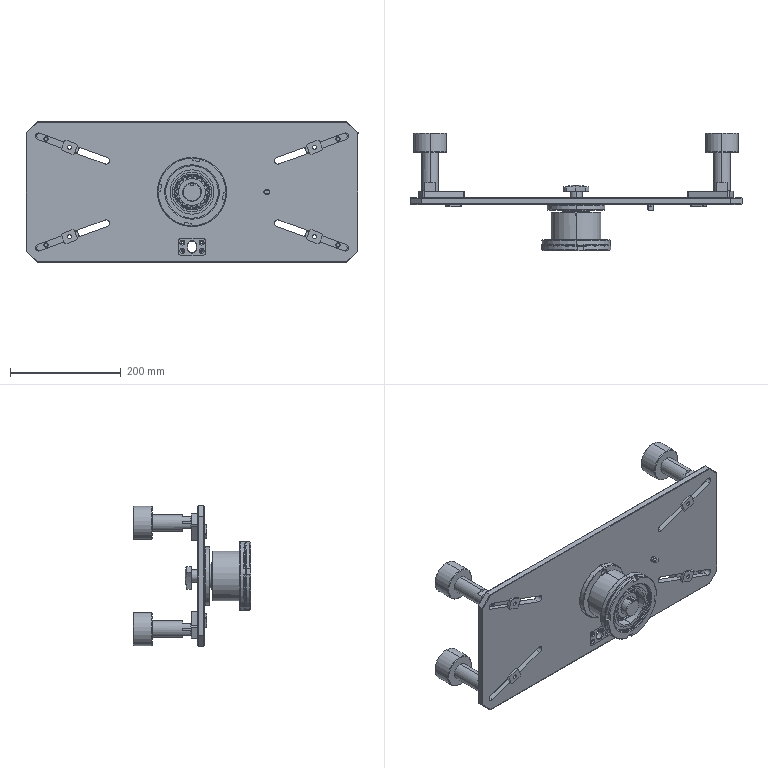Assembly | SolidWorks | mm | 30 component files | 30 solids | 1128 faces | box 600 x 213 x 255 mm | volume 2843561 mm3 | plane 427 | cone 266 | cylinder 261 | torus 164 | spline 10 | commonest cylinder face diameters 10 x25 8.5 x20 15 x16 8 x16 6.8 x16 12 x12 6 x9 16 x9
Bill of materials:
JBH10-8 | 2 | '- | Flanged cylindrical sleeve with a plain through bore; a short, wider flange at one end and a longer, smaller-diameter shank.
MA060.03.03-01 | 1 | AL5052 | Thin flat rectangular plate with chamfered corners, four long slots angled toward the corners, and a central group of round holes.
MA060.03.03-02 | 1 | 45# | Stepped turned pin: a small-diameter spigot, a larger cylindrical body, and a tapered conical nose with a rounded end.
MA060.03.03-03 | 1 | 45# | Flanged hub sleeve: a round flange with six bolt-circle holes, a large central bore with two opposite keyway-like notches, and a cylindrical sleeve with a small V-notch at its end.
MA060.03.03-04 | 1 | 45# | Flanged stub shaft: a round flange with holes, short bosses on both faces, and a stepped shaft with a groove and an end slot or keyway.
MA060.03.03-05 | 1 | 45# | Hexagonal-bodied stepped stud: a small cylindrical spigot with a bore, a hexagonal body, and a tapered, rounded nose.
MA060.03.03-06 | 4 | Q235A | Elongated rectangular bar with chamfered corners, two round through holes, and a stepped (offset-layer) cross-section.
MA060.03.03-07 | 4 | Q235A | Small rectangular block with chamfered corners, a single central through hole, and a stepped, two-tier profile.
MA060.03.03-08 | 1 | H68 | Rectangular flange plate with rounded corners, four countersunk holes, and a central obround opening surrounded by a raised obround boss.
MA060.03.03-09 | 1 | Q235A | Cylindrical pin with two parallel flats machined along part of its length, forming a reduced flat-sided end section.
MA060.03.03-10 | 4 | Polyurethane | Solid cylindrical disc or spacer with a small central through hole and chamfered edges.
MA060.03.03-11 | 4 | Chrome Plated Round Bar | Stepped cylindrical pin: a large cylindrical body with a flat-sided reduced section at one end and a small-diameter pin projecting from that end.
NTM10-30 | 1 | '- | Hand-knob-like part: three-lobed head with concave sides and a slightly domed top face, with a cylindrical shoulder and then a smaller plain cylindrical shank with a chamfered end, all on one axis.
small round nuts gb | 1 |  | Thin flat annular ring with four evenly spaced rectangular notches around the outside and chamfered edges; looks like a slotted ring nut.
tab washers for round nut gb | 1 |  | Thin washer-like ring with one inward rectangular tab and six outward rectangular tabs in two groups of three. The outer tabs are bent out of the plane of the ring at different angles. It looks like a tab-style locking washer.
tapered roller bearings gb | 2 |  | Rolling-element bearing-like assembly: an outer ring and an inner ring with a ring of round rolling elements packed closely between them. The inner ring sticks out past the outer ring on one face.
Mates:
1. coincident | MA060.03.03-03-1 plane at (0, 0, 0) dir (0, 0, 1) | assembly plane at (0, 0, 0) dir (0, 0, 1)
2. coincident | MA060.03.03-03-1 plane at (0, 0, 0) dir (0, 1, 0) | assembly plane at (0, 0, 0) dir (0, 1, 0)
3. coincident | MA060.03.03-03-1 plane at (0, 0, 0) dir (1, 0, 0) | assembly plane at (0, 0, 0) dir (1, 0, 0)
4. concentric | MA060.03.03-04-1 face at (0, 80.553, 0) dir (0, -1, 0) r 25 | MA060.03.03-01-1 face at (0, 81.053, 0) dir (0, -1, 0) r 25
5. coincident | MA060.03.03-04-1 face at (0, 78.053, 0) dir (0, 1, 0) | MA060.03.03-01-1 face at (0, 78.053, 0) dir (0, -1, 0)
6. concentric | MA060.03.03-01-1 face at (0, 78.053, -99) dir (0, 1, 0) r 12.5 | MA060.03.03-08-1 face at (0, 90.053, -99) dir (0, -1, 0) r 12.5
7. coincident | MA060.03.03-01-1 face at (0, 83.053, 0) dir (0, -1, 0) | MA060.03.03-08-1 face at (0, 83.053, -99) dir (0, 1, 0)
8. concentric | MA060.03.03-01-1 face at (17.5, 83.053, -106.5) dir (0, -1, 0) r 1.65 | MA060.03.03-08-1 face at (17.5, 78.053, -106.5) dir (0, -1, 0) r 2.25
9. parallel | MA060.03.03-01-1 face at (300, 78.053, -127.5) dir (0, 0, -1) | assembly plane at (0, 0, 0) dir (0, 0, 1)
10. coincident | MA060.03.03-01-1 face at (-275.157, 78.053, -106.534) dir (-0.342, 0, 0.9397) | MA060.03.03-06-2 face at (-278.591, 87.053, -107.784) dir (0.342, 0, -0.9397)
11. coincident | MA060.03.03-01-1 face at (0, 90.053, 0) dir (0, 1, 0) | MA060.03.03-06-2 face at (-276.35, 90.053, -113.939) dir (0, -1, 0)
12. concentric | MA060.03.03-07-9 face at (-221.425, 74.053, -80.645) dir (0, -1, 0) r 3.4 | MA060.03.03-06-2 face at (-221.425, 87.053, -80.645) dir (0, 1, 0) r 4.25
13. coincident | MA060.03.03-01-1 face at (0, 78.053, 0) dir (0, -1, 0) | MA060.03.03-07-9 face at (-213.099, 78.053, -66.973) dir (0, 1, 0)
14. parallel | MA060.03.03-01-1 face at (-275.157, 78.053, -106.534) dir (-0.342, 0, 0.9397) | MA060.03.03-07-9 face at (-213.099, 74.053, -66.973) dir (-0.342, 0, 0.9397)
15. concentric | MA060.03.03-01-1 face at (-41, 90.053, 0) dir (0, 1, 0) r 7.5 | JBH10-8-1 face at (-41, 85.753, 0) dir (0, 1, 0) r 7.5
16. coincident | MA060.03.03-01-1 face at (-41, 82.253, 0) dir (0, -1, 0) | JBH10-8-1 face at (-49.75, 82.253, 0) dir (0, 1, 0)
17. concentric | MA060.03.03-04-1 face at (-41, 72.053, 0) dir (0, 1, 0) r 3 | MA060.03.03-02-1 face at (-41, 73.053, 0) dir (0, -1, 0) r 3
18. coincident | MA060.03.03-04-1 face at (0, 78.053, 0) dir (0, 1, 0) | MA060.03.03-02-1 face at (-36, 78.053, 0) dir (0, -1, 0)
19. coincident | MA060.03.03-04-1 face at (0, 78.053, 0) dir (0, 1, 0) | MA060.03.03-05-2 face at (46, 78.053, 0) dir (0, -1, 0)
20. concentric | MA060.03.03-04-1 face at (41, 72.053, 0) dir (0, 1, 0) r 3 | MA060.03.03-05-2 face at (41, 73.053, 0) dir (0, -1, 0) r 3
21. concentric | MA060.03.03-01-1 face at (0, 78.053, 0) dir (0, 1, 0) r 5.5 | NTM10-30-1 face at (0, 75.513, 0) dir (0, -1, 0) r 5
22. coincident | MA060.03.03-01-1 face at (0, 90.053, 0) dir (0, 1, 0) | NTM10-30-1 face at (5.5, 90.053, 0) dir (0, -1, 0)
23. coincident | MA060.03.03-01-1 face at (132.25, 86.053, 0) dir (0, -1, 0) | MA060.03.03-09-11 face at (135, 86.053, 0) dir (0, 1, 0)
24. concentric | MA060.03.03-01-1 face at (135, 78.053, 0) dir (0, -1, 0) r 5 | MA060.03.03-09-11 face at (135, 68.053, 0) dir (0, -1, 0) r 5
25. parallel | MA060.03.03-01-1 face at (300, 78.053, 127.5) dir (0, 0, 1) | MA060.03.03-09-11 face at (139.33, 78.053, 2.5) dir (0, 0, 1)
26. concentric | MA060.03.03-06-2 face at (-263.711, 102.053, -96.036) dir (0, 1, 0) r 4 | MA060.03.03-10-2 face at (-263.711, 207.053, -96.036) dir (0, 1, 0) r 4.5
27. distance | MA060.03.03-06-2 face at (-243.038, 102.053, -88.512) dir (0, 1, 0) | MA060.03.03-10-2 face at (-263.711, 172.053, -96.036) dir (0, -1, 0)
28. concentric | MA060.03.03-10-2 face at (-263.711, 172.053, -96.036) dir (0, -1, 0) r 30 | MA060.03.03-11-2 face at (-263.711, 188.391, -96.036) dir (0, 1, 0) r 15
29. coincident | MA060.03.03-10-2 face at (-263.711, 172.053, -96.036) dir (0, -1, 0) | MA060.03.03-11-2 face at (-263.711, 172.053, -96.036) dir (0, 1, 0)
30. coincident | MA060.03.03-03-1 face at (32.5, 26, 0) dir (0, -1, 0) | tapered roller bearings gb-2 face at (16.537, 26, 26.81) dir (0, 1, 0)
31. concentric | MA060.03.03-03-1 face at (0, 0, 0) dir (0, -1, 0) r 36 | tapered roller bearings gb-2 face at (0, 7.747, 0) dir (0, 1, 0) r 32.5
32. coincident | MA060.03.03-03-1 face at (36, 46.5, 0) dir (0, 1, 0) | tapered roller bearings gb-3 face at (-2.815, 46.5, 31.374) dir (0, -1, 0)
33. concentric | MA060.03.03-04-1 face at (0, 64.753, 0) dir (0, -1, 0) r 17.5 | tapered roller bearings gb-3 face at (0, 64.753, 0) dir (0, -1, 0) r 32.5
34. coincident | MA060.03.03-04-1 face at (0, 64.753, 0) dir (0, -1, 0) | tapered roller bearings gb-3 face at (0, 64.753, 0) dir (0, 1, 0)
35. coincident | tapered roller bearings gb-2 face at (0, 7.747, 0) dir (0, -1, 0) | tab washers for round nut gb-1 face at (0, 7.747, 0) dir (0, 1, 0)
36. concentric | MA060.03.03-04-1 face at (0, 12.053, 0) dir (0, -1, 0) r 16.5 | tab washers for round nut gb-1 face at (0, 4.838, 0) dir (0, 1, 0) r 5.25
37. concentric | MA060.03.03-04-1 face at (0, 12.053, 0) dir (0, -1, 0) r 16.5 | NTM10-30-1 face at (0, 96.053, 0) dir (0, -1, 0) r 11
38. concentric | MA060.03.03-04-1 face at (0, 12.053, 0) dir (0, -1, 0) r 16.5 | tapered roller bearings gb-2 face at (0, 7.747, 0) dir (0, 1, 0) r 16
39. parallel | MA060.03.03-01-1 face at (300, 78.053, 127.5) dir (1, 0, 0) | MA060.03.03-04-1 face at (-3, 12.053, 44.5) dir (1, 0, 0)
40. parallel | MA060.03.03-04-1 face at (-3, 12.053, 44.5) dir (1, 0, 0) | tab washers for round nut gb-1 face at (-1.9, 4.838, 4.894) dir (-1, 0, 0)
41. coincident | small round nuts gb-1 face at (0, 6.747, 0) dir (0, 1, 0) | tab washers for round nut gb-1 face at (8, 6.747, 0) dir (0, -1, 0)
42. concentric | MA060.03.03-04-1 face at (0, 12.053, 0) dir (0, -1, 0) r 16.5 | small round nuts gb-1 face at (0, -5.253, 0) dir (0, 1, 0) r 47.5